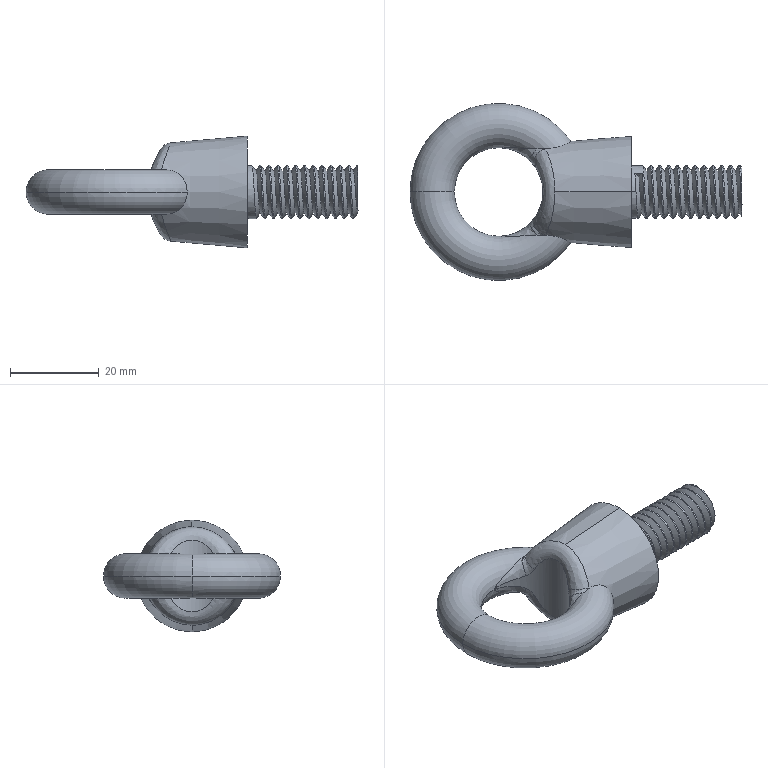Component | SolidWorks | M12LiftingEye-1 | 1 solid | 48 faces | volume 17020 mm3 | cylinder 26 | spline 12 | torus 4 | plane 4 | cone 2 | commonest cylinder face diameters 12 x25 20 x1